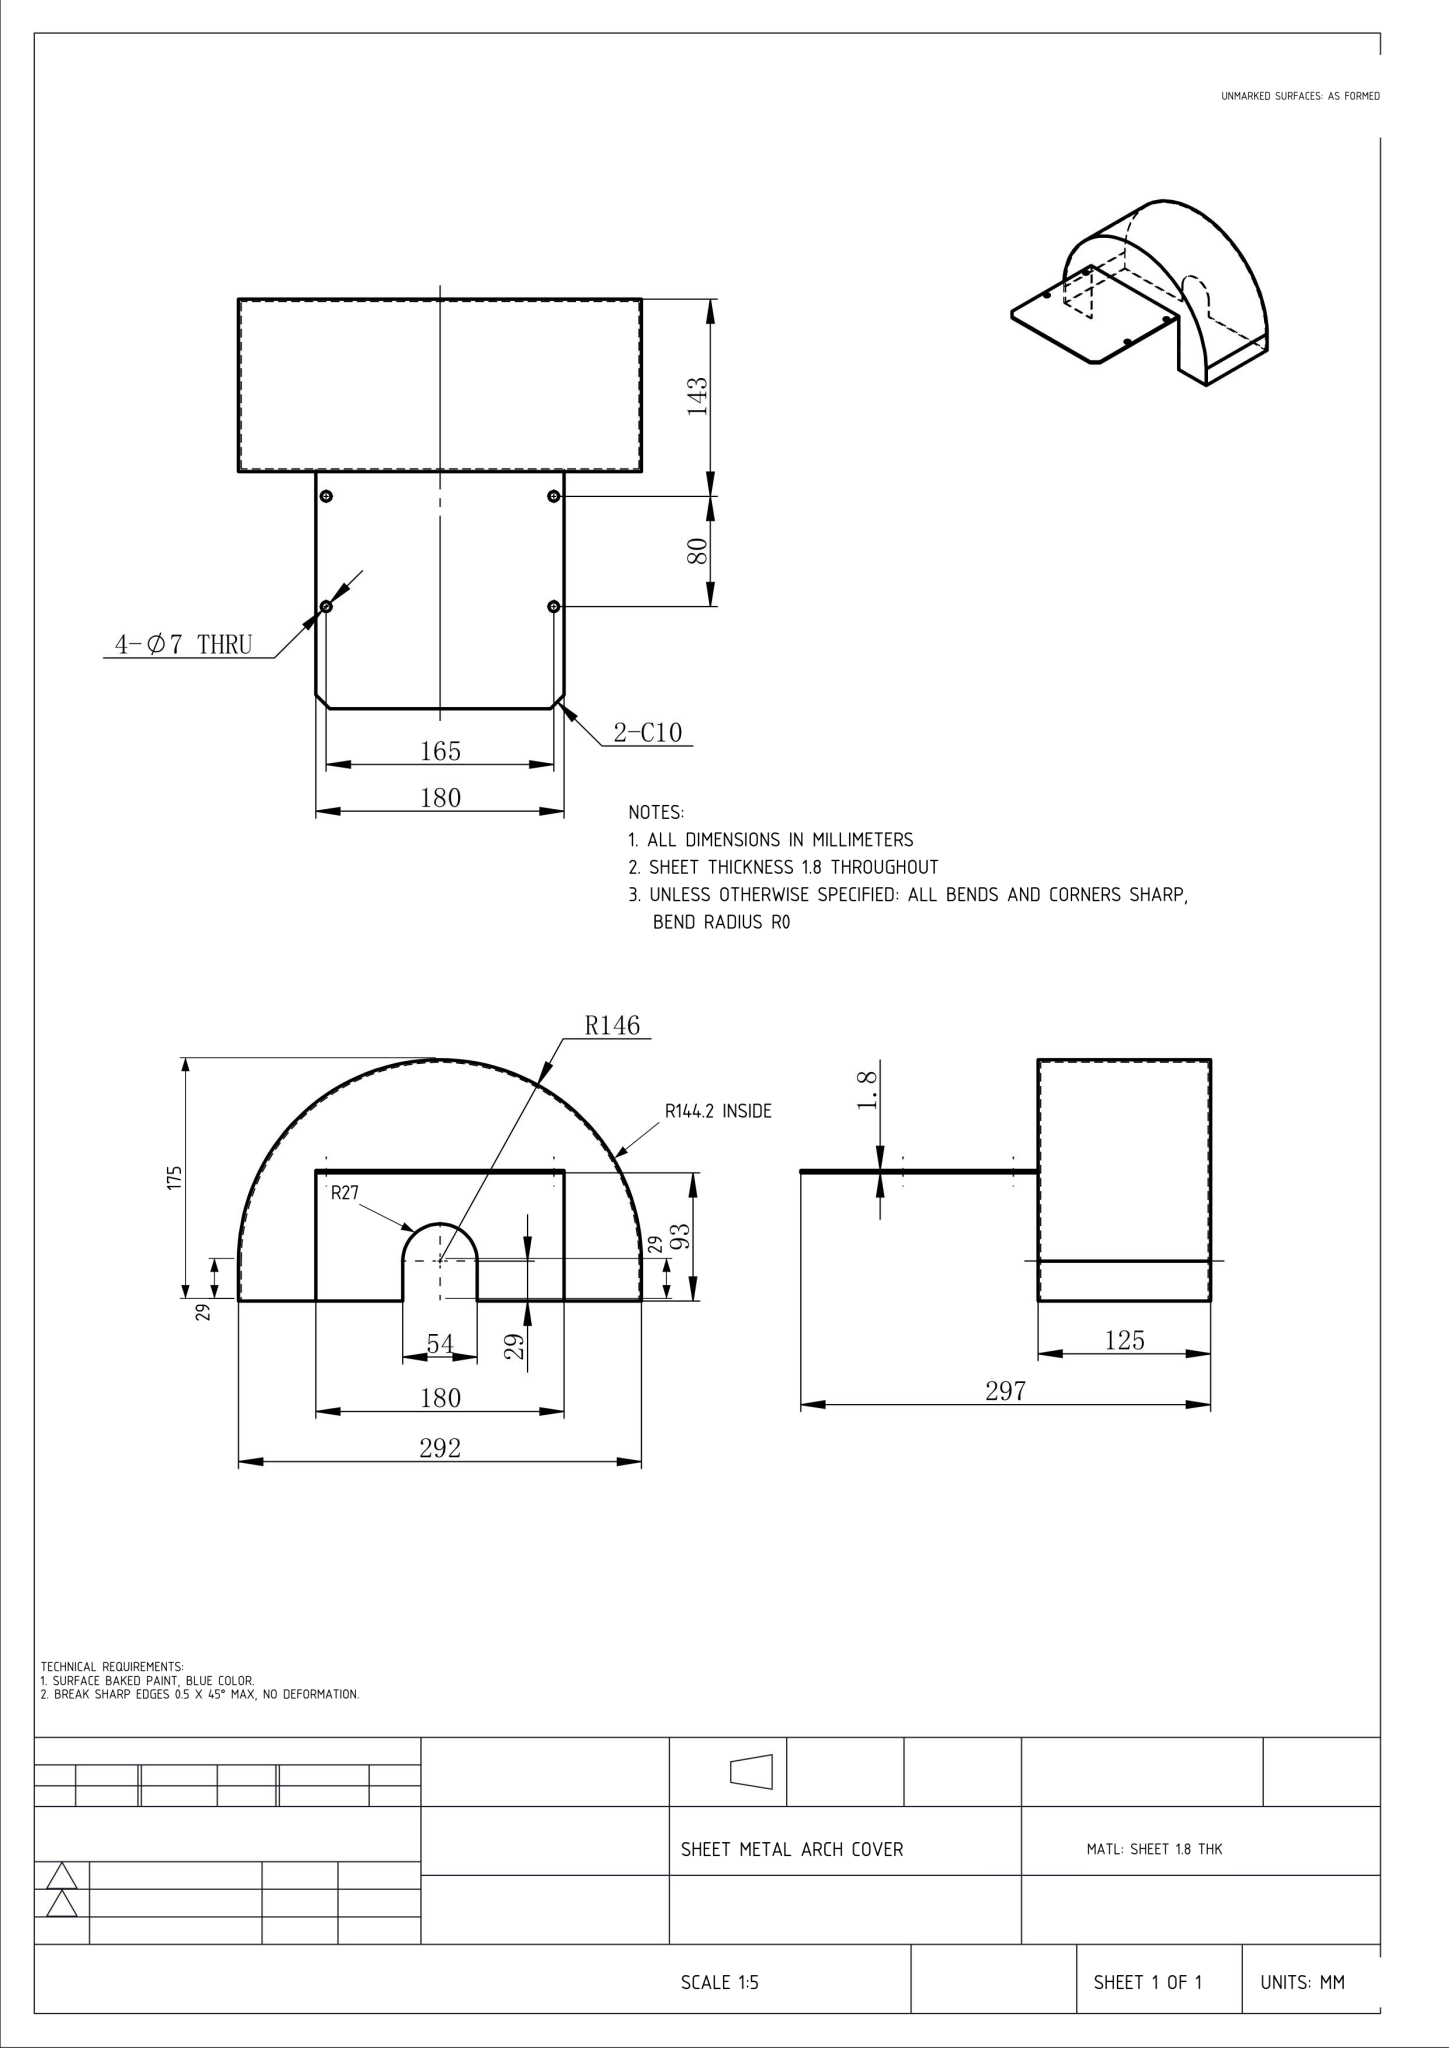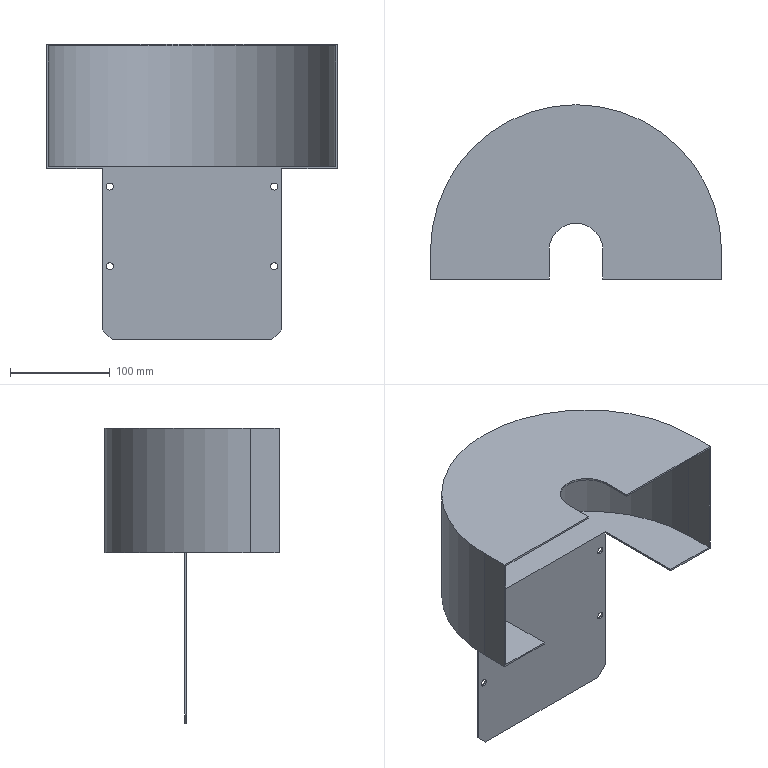Part | NX | mm | 1 solid | 32 faces | box 292 x 175 x 297 mm | volume 283568 mm3 | plane 21 | cylinder 11 | commonest cylinder face diameters 7 x8 288.4 x1 292 x1 54 x1